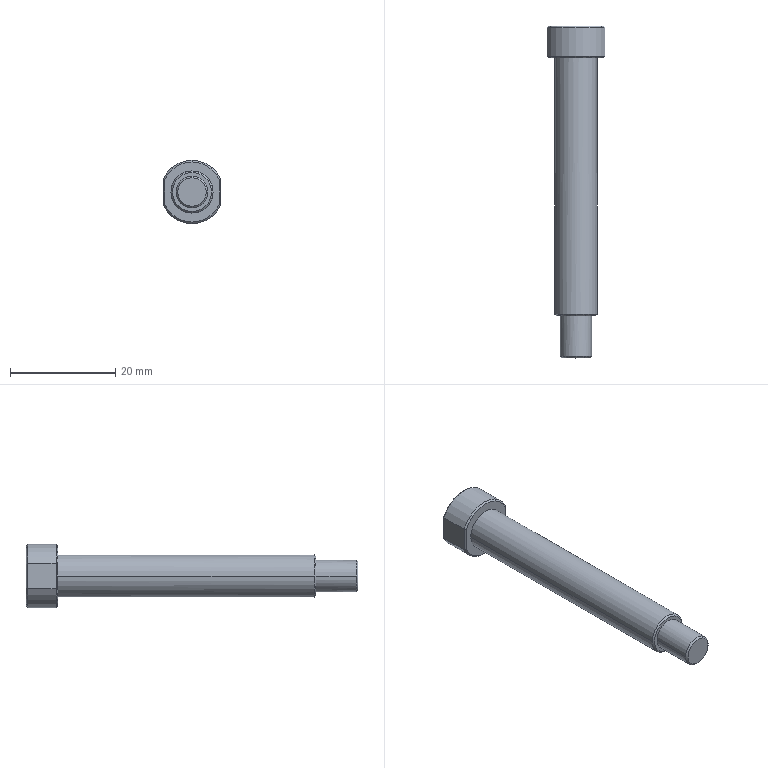Component | SolidWorks | LH-CGJ-01-058-2 | 1 solid | 26 faces | box 11 x 63 x 12 mm | volume 3343 mm3 | cone 10 | plane 10 | cylinder 6 | commonest cylinder face diameters 8 x2 6 x2 12 x2 | material #45
build123d program:
from build123d import *

# Parameters (mm, degrees)
CUT_EXTRUDE1_DEPTH = 59.558
CHAMFER1_SIZE      = 0.3


with BuildPart() as part:
    # Sketch1 → Revolve2 (revolve)
    with BuildSketch(Plane.XY, mode=Mode.PRIVATE) as revolve2_sk:
        Polygon((0, 0), (6, 0), (6, -63), (3, -63), (3, -55), (2, -55), (2, -6), (0, -6), align=None)
    revolve(revolve2_sk.sketch.rotate(Axis((6, -63, 0), (0, 1, 0)), 180), axis=Axis((6, -63, 0), (0, 1, 0)))

    # Sketch2 → Cut-Extrude1 (cut, through all)
    with BuildSketch(Plane.XZ.offset(6)):
        with BuildLine():
            Line((0.5, 2.398), (0.5, -2.398))
            ThreePointArc((0.5, -2.398), (0, 0), (0.5, 2.398))
        make_face()
        with BuildLine():
            Line((11.5, 2.398), (11.5, -2.398))
            ThreePointArc((11.5, -2.398), (12, 0), (11.5, 2.398))
        make_face()
    extrude(amount=-CUT_EXTRUDE1_DEPTH, mode=Mode.SUBTRACT)

    # Chamfer1
    chamfer1_edges = [part.edges().sort_by_distance(p)[0] for p in [
        (6, -6, -6),
        (6, 0, -6),
        (11.5, 0, 0),
        (11.5, -6, 0),
        (0.5, 0, 0),
        (0.5, -6, 0),
        (6, -6, 6),
        (2, -55, 0),
        (3, -63, 0),
        (6, 0, 6),
    ]]
    chamfer(chamfer1_edges, length=CHAMFER1_SIZE)


solid = part.part

# Placed as in the assembly
solid = solid.moved(Location((-42.003, 46.715, 115.05), (0, 0, 0)))
STEP:
#1=COLOUR_RGB('',0.7922,0.8196,0.9333);
#2=FILL_AREA_STYLE_COLOUR('',#1);
#3=FILL_AREA_STYLE('',(#2));
#4=SURFACE_STYLE_FILL_AREA(#3);
#5=SURFACE_SIDE_STYLE('',(#4));
#6=SURFACE_STYLE_USAGE(.BOTH.,#5);
#7=PRESENTATION_STYLE_ASSIGNMENT((#6));
#8=CARTESIAN_POINT('',(-1.417,-0.3262,4.384));
#9=VERTEX_POINT('',#8);
#10=CARTESIAN_POINT('',(-1.417,-0.3262,4.675));
#11=VERTEX_POINT('',#10);
#12=CARTESIAN_POINT('',(-1.417,-0.3262,4.53));
#13=DIRECTION('',(-0.,-1.,0.));
#14=DIRECTION('',(-1.,0.,0.));
#15=AXIS2_PLACEMENT_3D('',#12,#13,#14);
#16=CIRCLE('',#15,0.1457);
#17=EDGE_CURVE('',#9,#11,#16,.T.);
#18=ORIENTED_EDGE('',*,*,#17,.F.);
#19=CARTESIAN_POINT('',(-1.417,-0.3144,4.372));
#20=VERTEX_POINT('',#19);
#21=CARTESIAN_POINT('',(-1.417,-0.3262,4.384));
#22=DIRECTION('',(0.,0.7071,-0.7071));
#23=VECTOR('',#22,39.37);
#24=LINE('',#21,#23);
#25=EDGE_CURVE('',#9,#20,#24,.T.);
#26=ORIENTED_EDGE('',*,*,#25,.T.);
#27=CARTESIAN_POINT('',(-1.26,-0.3144,4.53));
#28=VERTEX_POINT('',#27);
#29=CARTESIAN_POINT('',(-1.417,-0.3144,4.53));
#30=DIRECTION('',(0.,1.,0.));
#31=DIRECTION('',(0.,0.,1.));
#32=AXIS2_PLACEMENT_3D('',#29,#30,#31);
#33=CIRCLE('',#32,0.1575);
#34=EDGE_CURVE('',#28,#20,#33,.T.);
#35=ORIENTED_EDGE('',*,*,#34,.F.);
#36=CARTESIAN_POINT('',(-1.417,-0.3144,4.687));
#37=VERTEX_POINT('',#36);
#38=CARTESIAN_POINT('',(-1.417,-0.3144,4.53));
#39=DIRECTION('',(0.,1.,0.));
#40=DIRECTION('',(0.,0.,1.));
#41=AXIS2_PLACEMENT_3D('',#38,#39,#40);
#42=CIRCLE('',#41,0.1575);
#43=EDGE_CURVE('',#37,#28,#42,.T.);
#44=ORIENTED_EDGE('',*,*,#43,.F.);
#45=CARTESIAN_POINT('',(-1.417,-0.3262,4.675));
#46=DIRECTION('',(0.,0.7071,0.7071));
#47=VECTOR('',#46,39.37);
#48=LINE('',#45,#47);
#49=EDGE_CURVE('',#11,#37,#48,.T.);
#50=ORIENTED_EDGE('',*,*,#49,.F.);
#51=EDGE_LOOP('',(#18,#26,#35,#44,#50));
#52=FACE_OUTER_BOUND('',#51,.T.);
#53=CARTESIAN_POINT('',(-1.417,-0.3262,4.53));
#54=DIRECTION('',(0.,1.,0.));
#55=DIRECTION('',(0.,0.,1.));
#56=AXIS2_PLACEMENT_3D('',#53,#54,#55);
#57=CONICAL_SURFACE('',#56,0.1457,0.7854);
#58=ADVANCED_FACE('',(#52),#57,.T.);
#59=CARTESIAN_POINT('',(-1.417,-0.6411,4.423));
#60=VERTEX_POINT('',#59);
#61=CARTESIAN_POINT('',(-1.417,-0.6411,4.636));
#62=VERTEX_POINT('',#61);
#63=CARTESIAN_POINT('',(-1.417,-0.6411,4.53));
#64=DIRECTION('',(-0.,-1.,0.));
#65=DIRECTION('',(-1.,0.,0.));
#66=AXIS2_PLACEMENT_3D('',#63,#64,#65);
#67=CIRCLE('',#66,0.1063);
#68=EDGE_CURVE('',#60,#62,#67,.T.);
#69=ORIENTED_EDGE('',*,*,#68,.F.);
#70=CARTESIAN_POINT('',(-1.417,-0.6293,4.411));
#71=VERTEX_POINT('',#70);
#72=CARTESIAN_POINT('',(-1.417,-0.6411,4.423));
#73=DIRECTION('',(0.,0.7071,-0.7071));
#74=VECTOR('',#73,39.37);
#75=LINE('',#72,#74);
#76=EDGE_CURVE('',#60,#71,#75,.T.);
#77=ORIENTED_EDGE('',*,*,#76,.T.);
#78=CARTESIAN_POINT('',(-1.299,-0.6293,4.53));
#79=VERTEX_POINT('',#78);
#80=CARTESIAN_POINT('',(-1.417,-0.6293,4.53));
#81=DIRECTION('',(0.,1.,0.));
#82=DIRECTION('',(0.,0.,1.));
#83=AXIS2_PLACEMENT_3D('',#80,#81,#82);
#84=CIRCLE('',#83,0.1181);
#85=EDGE_CURVE('',#79,#71,#84,.T.);
#86=ORIENTED_EDGE('',*,*,#85,.F.);
#87=CARTESIAN_POINT('',(-1.417,-0.6293,4.648));
#88=VERTEX_POINT('',#87);
#89=CARTESIAN_POINT('',(-1.417,-0.6293,4.53));
#90=DIRECTION('',(0.,1.,0.));
#91=DIRECTION('',(0.,0.,1.));
#92=AXIS2_PLACEMENT_3D('',#89,#90,#91);
#93=CIRCLE('',#92,0.1181);
#94=EDGE_CURVE('',#88,#79,#93,.T.);
#95=ORIENTED_EDGE('',*,*,#94,.F.);
#96=CARTESIAN_POINT('',(-1.417,-0.6411,4.636));
#97=DIRECTION('',(0.,0.7071,0.7071));
#98=VECTOR('',#97,39.37);
#99=LINE('',#96,#98);
#100=EDGE_CURVE('',#62,#88,#99,.T.);
#101=ORIENTED_EDGE('',*,*,#100,.F.);
#102=EDGE_LOOP('',(#69,#77,#86,#95,#101));
#103=FACE_OUTER_BOUND('',#102,.T.);
#104=CARTESIAN_POINT('',(-1.417,-0.6411,4.53));
#105=DIRECTION('',(0.,1.,0.));
#106=DIRECTION('',(0.,0.,1.));
#107=AXIS2_PLACEMENT_3D('',#104,#105,#106);
#108=CONICAL_SURFACE('',#107,0.1063,0.7854);
#109=ADVANCED_FACE('',(#103),#108,.T.);
#110=CARTESIAN_POINT('',(-1.417,1.603,4.754));
#111=VERTEX_POINT('',#110);
#112=CARTESIAN_POINT('',(-1.622,1.603,4.621));
#113=VERTEX_POINT('',#112);
#114=CARTESIAN_POINT('',(-1.417,1.603,4.53));
#115=DIRECTION('',(-0.,-1.,0.));
#116=DIRECTION('',(-1.,0.,0.));
#117=AXIS2_PLACEMENT_3D('',#114,#115,#116);
#118=CIRCLE('',#117,0.2244);
#119=EDGE_CURVE('',#111,#113,#118,.T.);
#120=ORIENTED_EDGE('',*,*,#119,.F.);
#121=CARTESIAN_POINT('',(-1.417,1.615,4.766));
#122=VERTEX_POINT('',#121);
#123=CARTESIAN_POINT('',(-1.417,1.603,4.754));
#124=DIRECTION('',(0.,0.7071,0.7071));
#125=VECTOR('',#124,39.37);
#126=LINE('',#123,#125);
#127=EDGE_CURVE('',#111,#122,#126,.T.);
#128=ORIENTED_EDGE('',*,*,#127,.T.);
#129=CARTESIAN_POINT('',(-1.634,1.615,4.624));
#130=VERTEX_POINT('',#129);
#131=CARTESIAN_POINT('',(-1.417,1.615,4.53));
#132=DIRECTION('',(0.,1.,0.));
#133=DIRECTION('',(0.,0.,1.));
#134=AXIS2_PLACEMENT_3D('',#131,#132,#133);
#135=CIRCLE('',#134,0.2362);
#136=EDGE_CURVE('',#130,#122,#135,.T.);
#137=ORIENTED_EDGE('',*,*,#136,.F.);
#138=CARTESIAN_POINT('',(-1.634,1.615,4.624));
#139=CARTESIAN_POINT('',(-1.63,1.611,4.623));
#140=CARTESIAN_POINT('',(-1.626,1.607,4.622));
#141=CARTESIAN_POINT('',(-1.622,1.603,4.621));
#142=B_SPLINE_CURVE_WITH_KNOTS('',3,(#138,#139,#140,#141),.UNSPECIFIED.,.F.,.F.,(4,4),(0.,0.000429),.UNSPECIFIED.);
#143=EDGE_CURVE('',#130,#113,#142,.T.);
#144=ORIENTED_EDGE('',*,*,#143,.T.);
#145=EDGE_LOOP('',(#120,#128,#137,#144));
#146=FACE_OUTER_BOUND('',#145,.T.);
#147=CARTESIAN_POINT('',(-1.417,1.603,4.53));
#148=DIRECTION('',(0.,1.,0.));
#149=DIRECTION('',(0.,0.,1.));
#150=AXIS2_PLACEMENT_3D('',#147,#148,#149);
#151=CONICAL_SURFACE('',#150,0.2244,0.7854);
#152=ADVANCED_FACE('',(#146),#151,.T.);
#153=CARTESIAN_POINT('',(-1.417,1.839,4.305));
#154=VERTEX_POINT('',#153);
#155=CARTESIAN_POINT('',(-1.622,1.839,4.438));
#156=VERTEX_POINT('',#155);
#157=CARTESIAN_POINT('',(-1.417,1.839,4.53));
#158=DIRECTION('',(0.,1.,0.));
#159=DIRECTION('',(1.,0.,0.));
#160=AXIS2_PLACEMENT_3D('',#157,#158,#159);
#161=CIRCLE('',#160,0.2244);
#162=EDGE_CURVE('',#154,#156,#161,.T.);
#163=ORIENTED_EDGE('',*,*,#162,.F.);
#164=CARTESIAN_POINT('',(-1.417,1.827,4.293));
#165=VERTEX_POINT('',#164);
#166=CARTESIAN_POINT('',(-1.417,1.827,4.293));
#167=DIRECTION('',(0.,-0.7071,-0.7071));
#168=VECTOR('',#167,39.37);
#169=LINE('',#166,#168);
#170=EDGE_CURVE('',#154,#165,#169,.T.);
#171=ORIENTED_EDGE('',*,*,#170,.T.);
#172=CARTESIAN_POINT('',(-1.634,1.827,4.435));
#173=VERTEX_POINT('',#172);
#174=CARTESIAN_POINT('',(-1.417,1.827,4.53));
#175=DIRECTION('',(0.,-1.,0.));
#176=DIRECTION('',(0.,0.,-1.));
#177=AXIS2_PLACEMENT_3D('',#174,#175,#176);
#178=CIRCLE('',#177,0.2362);
#179=EDGE_CURVE('',#173,#165,#178,.T.);
#180=ORIENTED_EDGE('',*,*,#179,.F.);
#181=CARTESIAN_POINT('',(-1.622,1.839,4.438));
#182=CARTESIAN_POINT('',(-1.626,1.835,4.437));
#183=CARTESIAN_POINT('',(-1.63,1.831,4.436));
#184=CARTESIAN_POINT('',(-1.634,1.827,4.435));
#185=B_SPLINE_CURVE_WITH_KNOTS('',3,(#181,#182,#183,#184),.UNSPECIFIED.,.F.,.F.,(4,4),(0.,0.000429),.UNSPECIFIED.);
#186=EDGE_CURVE('',#156,#173,#185,.T.);
#187=ORIENTED_EDGE('',*,*,#186,.F.);
#188=EDGE_LOOP('',(#163,#171,#180,#187));
#189=FACE_OUTER_BOUND('',#188,.T.);
#190=CARTESIAN_POINT('',(-1.417,1.827,4.53));
#191=DIRECTION('',(0.,-1.,0.));
#192=DIRECTION('',(0.,0.,-1.));
#193=AXIS2_PLACEMENT_3D('',#190,#191,#192);
#194=CONICAL_SURFACE('',#193,0.2362,0.7854);
#195=ADVANCED_FACE('',(#189),#194,.T.);
#196=CARTESIAN_POINT('',(-1.26,1.603,4.53));
#197=VERTEX_POINT('',#196);
#198=CARTESIAN_POINT('',(-1.575,1.603,4.53));
#199=VERTEX_POINT('',#198);
#200=CARTESIAN_POINT('',(-1.417,1.603,4.53));
#201=DIRECTION('',(-0.,-1.,0.));
#202=DIRECTION('',(1.,0.,0.));
#203=AXIS2_PLACEMENT_3D('',#200,#201,#202);
#204=CIRCLE('',#203,0.1575);
#205=EDGE_CURVE('',#197,#199,#204,.T.);
#206=ORIENTED_EDGE('',*,*,#205,.T.);
#207=CARTESIAN_POINT('',(-1.575,-0.3144,4.53));
#208=VERTEX_POINT('',#207);
#209=CARTESIAN_POINT('',(-1.575,-0.6411,4.53));
#210=DIRECTION('',(-0.,-1.,0.));
#211=VECTOR('',#210,39.37);
#212=LINE('',#209,#211);
#213=EDGE_CURVE('',#199,#208,#212,.T.);
#214=ORIENTED_EDGE('',*,*,#213,.T.);
#215=CARTESIAN_POINT('',(-1.417,-0.3144,4.53));
#216=DIRECTION('',(0.,1.,0.));
#217=DIRECTION('',(0.,0.,1.));
#218=AXIS2_PLACEMENT_3D('',#215,#216,#217);
#219=CIRCLE('',#218,0.1575);
#220=EDGE_CURVE('',#208,#37,#219,.T.);
#221=ORIENTED_EDGE('',*,*,#220,.T.);
#222=ORIENTED_EDGE('',*,*,#43,.T.);
#223=CARTESIAN_POINT('',(-1.26,-0.6411,4.53));
#224=DIRECTION('',(-0.,-1.,0.));
#225=VECTOR('',#224,39.37);
#226=LINE('',#223,#225);
#227=EDGE_CURVE('',#197,#28,#226,.T.);
#228=ORIENTED_EDGE('',*,*,#227,.F.);
#229=EDGE_LOOP('',(#206,#214,#221,#222,#228));
#230=FACE_OUTER_BOUND('',#229,.T.);
#231=CARTESIAN_POINT('',(-1.417,-0.6411,4.53));
#232=DIRECTION('',(-0.,-1.,0.));
#233=DIRECTION('',(1.,0.,0.));
#234=AXIS2_PLACEMENT_3D('',#231,#232,#233);
#235=CYLINDRICAL_SURFACE('',#234,0.1575);
#236=ADVANCED_FACE('',(#230),#235,.T.);
#237=CARTESIAN_POINT('',(-1.299,-0.3262,4.53));
#238=VERTEX_POINT('',#237);
#239=CARTESIAN_POINT('',(-1.536,-0.3262,4.53));
#240=VERTEX_POINT('',#239);
#241=CARTESIAN_POINT('',(-1.417,-0.3262,4.53));
#242=DIRECTION('',(-0.,-1.,0.));
#243=DIRECTION('',(1.,0.,0.));
#244=AXIS2_PLACEMENT_3D('',#241,#242,#243);
#245=CIRCLE('',#244,0.1181);
#246=EDGE_CURVE('',#238,#240,#245,.T.);
#247=ORIENTED_EDGE('',*,*,#246,.T.);
#248=CARTESIAN_POINT('',(-1.536,-0.6293,4.53));
#249=VERTEX_POINT('',#248);
#250=CARTESIAN_POINT('',(-1.536,-0.6411,4.53));
#251=DIRECTION('',(-0.,-1.,0.));
#252=VECTOR('',#251,39.37);
#253=LINE('',#250,#252);
#254=EDGE_CURVE('',#240,#249,#253,.T.);
#255=ORIENTED_EDGE('',*,*,#254,.T.);
#256=CARTESIAN_POINT('',(-1.417,-0.6293,4.53));
#257=DIRECTION('',(0.,1.,0.));
#258=DIRECTION('',(0.,0.,1.));
#259=AXIS2_PLACEMENT_3D('',#256,#257,#258);
#260=CIRCLE('',#259,0.1181);
#261=EDGE_CURVE('',#249,#88,#260,.T.);
#262=ORIENTED_EDGE('',*,*,#261,.T.);
#263=ORIENTED_EDGE('',*,*,#94,.T.);
#264=CARTESIAN_POINT('',(-1.299,-0.6411,4.53));
#265=DIRECTION('',(-0.,-1.,0.));
#266=VECTOR('',#265,39.37);
#267=LINE('',#264,#266);
#268=EDGE_CURVE('',#238,#79,#267,.T.);
#269=ORIENTED_EDGE('',*,*,#268,.F.);
#270=EDGE_LOOP('',(#247,#255,#262,#263,#269));
#271=FACE_OUTER_BOUND('',#270,.T.);
#272=CARTESIAN_POINT('',(-1.417,-0.6411,4.53));
#273=DIRECTION('',(-0.,-1.,0.));
#274=DIRECTION('',(1.,0.,0.));
#275=AXIS2_PLACEMENT_3D('',#272,#273,#274);
#276=CYLINDRICAL_SURFACE('',#275,0.1181);
#277=ADVANCED_FACE('',(#271),#276,.T.);
#278=CARTESIAN_POINT('',(-1.634,1.615,4.435));
#279=VERTEX_POINT('',#278);
#280=CARTESIAN_POINT('',(-1.634,1.839,4.435));
#281=DIRECTION('',(0.,-1.,0.));
#282=VECTOR('',#281,39.37);
#283=LINE('',#280,#282);
#284=EDGE_CURVE('',#173,#279,#283,.T.);
#285=ORIENTED_EDGE('',*,*,#284,.F.);
#286=ORIENTED_EDGE('',*,*,#179,.T.);
#287=CARTESIAN_POINT('',(-1.201,1.827,4.435));
#288=VERTEX_POINT('',#287);
#289=CARTESIAN_POINT('',(-1.417,1.827,4.53));
#290=DIRECTION('',(0.,-1.,0.));
#291=DIRECTION('',(0.,0.,-1.));
#292=AXIS2_PLACEMENT_3D('',#289,#290,#291);
#293=CIRCLE('',#292,0.2362);
#294=EDGE_CURVE('',#165,#288,#293,.T.);
#295=ORIENTED_EDGE('',*,*,#294,.T.);
#296=CARTESIAN_POINT('',(-1.201,1.615,4.435));
#297=VERTEX_POINT('',#296);
#298=CARTESIAN_POINT('',(-1.201,1.839,4.435));
#299=DIRECTION('',(0.,-1.,0.));
#300=VECTOR('',#299,39.37);
#301=LINE('',#298,#300);
#302=EDGE_CURVE('',#288,#297,#301,.T.);
#303=ORIENTED_EDGE('',*,*,#302,.T.);
#304=CARTESIAN_POINT('',(-1.417,1.615,4.53));
#305=DIRECTION('',(0.,1.,0.));
#306=DIRECTION('',(0.,0.,1.));
#307=AXIS2_PLACEMENT_3D('',#304,#305,#306);
#308=CIRCLE('',#307,0.2362);
#309=EDGE_CURVE('',#297,#279,#308,.T.);
#310=ORIENTED_EDGE('',*,*,#309,.T.);
#311=EDGE_LOOP('',(#285,#286,#295,#303,#310));
#312=FACE_OUTER_BOUND('',#311,.T.);
#313=CARTESIAN_POINT('',(-1.417,-0.6411,4.53));
#314=DIRECTION('',(-0.,-1.,0.));
#315=DIRECTION('',(1.,0.,0.));
#316=AXIS2_PLACEMENT_3D('',#313,#314,#315);
#317=CYLINDRICAL_SURFACE('',#316,0.2362);
#318=ADVANCED_FACE('',(#312),#317,.T.);
#319=CARTESIAN_POINT('',(-1.201,1.827,4.624));
#320=VERTEX_POINT('',#319);
#321=CARTESIAN_POINT('',(-1.201,1.615,4.624));
#322=VERTEX_POINT('',#321);
#323=CARTESIAN_POINT('',(-1.201,1.839,4.624));
#324=DIRECTION('',(0.,-1.,0.));
#325=VECTOR('',#324,39.37);
#326=LINE('',#323,#325);
#327=EDGE_CURVE('',#320,#322,#326,.T.);
#328=ORIENTED_EDGE('',*,*,#327,.F.);
#329=CARTESIAN_POINT('',(-1.634,1.827,4.624));
#330=VERTEX_POINT('',#329);
#331=CARTESIAN_POINT('',(-1.417,1.827,4.53));
#332=DIRECTION('',(0.,-1.,0.));
#333=DIRECTION('',(0.,0.,-1.));
#334=AXIS2_PLACEMENT_3D('',#331,#332,#333);
#335=CIRCLE('',#334,0.2362);
#336=EDGE_CURVE('',#320,#330,#335,.T.);
#337=ORIENTED_EDGE('',*,*,#336,.T.);
#338=CARTESIAN_POINT('',(-1.634,1.839,4.624));
#339=DIRECTION('',(0.,-1.,0.));
#340=VECTOR('',#339,39.37);
#341=LINE('',#338,#340);
#342=EDGE_CURVE('',#330,#130,#341,.T.);
#343=ORIENTED_EDGE('',*,*,#342,.T.);
#344=ORIENTED_EDGE('',*,*,#136,.T.);
#345=CARTESIAN_POINT('',(-1.417,1.615,4.53));
#346=DIRECTION('',(0.,1.,0.));
#347=DIRECTION('',(0.,0.,1.));
#348=AXIS2_PLACEMENT_3D('',#345,#346,#347);
#349=CIRCLE('',#348,0.2362);
#350=EDGE_CURVE('',#122,#322,#349,.T.);
#351=ORIENTED_EDGE('',*,*,#350,.T.);
#352=EDGE_LOOP('',(#328,#337,#343,#344,#351));
#353=FACE_OUTER_BOUND('',#352,.T.);
#354=CARTESIAN_POINT('',(-1.417,-0.6411,4.53));
#355=DIRECTION('',(-0.,-1.,0.));
#356=DIRECTION('',(1.,0.,0.));
#357=AXIS2_PLACEMENT_3D('',#354,#355,#356);
#358=CYLINDRICAL_SURFACE('',#357,0.2362);
#359=ADVANCED_FACE('',(#353),#358,.T.);
#360=CARTESIAN_POINT('',(-1.622,1.839,4.621));
#361=VERTEX_POINT('',#360);
#362=CARTESIAN_POINT('',(-1.622,1.839,4.53));
#363=DIRECTION('',(0.,0.,1.));
#364=VECTOR('',#363,39.37);
#365=LINE('',#362,#364);
#366=EDGE_CURVE('',#156,#361,#365,.T.);
#367=ORIENTED_EDGE('',*,*,#366,.T.);
#368=CARTESIAN_POINT('',(-1.213,1.839,4.621));
#369=VERTEX_POINT('',#368);
#370=CARTESIAN_POINT('',(-1.417,1.839,4.53));
#371=DIRECTION('',(0.,1.,0.));
#372=DIRECTION('',(1.,0.,0.));
#373=AXIS2_PLACEMENT_3D('',#370,#371,#372);
#374=CIRCLE('',#373,0.2244);
#375=EDGE_CURVE('',#361,#369,#374,.T.);
#376=ORIENTED_EDGE('',*,*,#375,.T.);
#377=CARTESIAN_POINT('',(-1.213,1.839,4.438));
#378=VERTEX_POINT('',#377);
#379=CARTESIAN_POINT('',(-1.213,1.839,4.53));
#380=DIRECTION('',(0.,0.,-1.));
#381=VECTOR('',#380,39.37);
#382=LINE('',#379,#381);
#383=EDGE_CURVE('',#369,#378,#382,.T.);
#384=ORIENTED_EDGE('',*,*,#383,.T.);
#385=CARTESIAN_POINT('',(-1.417,1.839,4.53));
#386=DIRECTION('',(0.,1.,0.));
#387=DIRECTION('',(1.,0.,0.));
#388=AXIS2_PLACEMENT_3D('',#385,#386,#387);
#389=CIRCLE('',#388,0.2244);
#390=EDGE_CURVE('',#378,#154,#389,.T.);
#391=ORIENTED_EDGE('',*,*,#390,.T.);
#392=ORIENTED_EDGE('',*,*,#162,.T.);
#393=EDGE_LOOP('',(#367,#376,#384,#391,#392));
#394=FACE_OUTER_BOUND('',#393,.T.);
#395=CARTESIAN_POINT('',(-1.654,1.839,4.53));
#396=DIRECTION('',(-0.,-1.,0.));
#397=DIRECTION('',(1.,-0.,0.));
#398=AXIS2_PLACEMENT_3D('',#395,#396,#397);
#399=PLANE('',#398);
#400=ADVANCED_FACE('',(#394),#399,.F.);
#401=CARTESIAN_POINT('',(-1.417,-0.6411,4.53));
#402=DIRECTION('',(-0.,-1.,0.));
#403=DIRECTION('',(-1.,0.,0.));
#404=AXIS2_PLACEMENT_3D('',#401,#402,#403);
#405=CIRCLE('',#404,0.1063);
#406=EDGE_CURVE('',#62,#60,#405,.T.);
#407=ORIENTED_EDGE('',*,*,#406,.T.);
#408=ORIENTED_EDGE('',*,*,#68,.T.);
#409=EDGE_LOOP('',(#407,#408));
#410=FACE_OUTER_BOUND('',#409,.T.);
#411=CARTESIAN_POINT('',(-1.417,-0.6411,4.53));
#412=DIRECTION('',(0.,1.,0.));
#413=DIRECTION('',(-1.,0.,0.));
#414=AXIS2_PLACEMENT_3D('',#411,#412,#413);
#415=PLANE('',#414);
#416=ADVANCED_FACE('',(#410),#415,.F.);
#417=ORIENTED_EDGE('',*,*,#254,.F.);
#418=CARTESIAN_POINT('',(-1.417,-0.3262,4.53));
#419=DIRECTION('',(-0.,-1.,0.));
#420=DIRECTION('',(1.,0.,0.));
#421=AXIS2_PLACEMENT_3D('',#418,#419,#420);
#422=CIRCLE('',#421,0.1181);
#423=EDGE_CURVE('',#240,#238,#422,.T.);
#424=ORIENTED_EDGE('',*,*,#423,.T.);
#425=ORIENTED_EDGE('',*,*,#268,.T.);
#426=ORIENTED_EDGE('',*,*,#85,.T.);
#427=CARTESIAN_POINT('',(-1.417,-0.6293,4.53));
#428=DIRECTION('',(0.,1.,0.));
#429=DIRECTION('',(0.,0.,1.));
#430=AXIS2_PLACEMENT_3D('',#427,#428,#429);
#431=CIRCLE('',#430,0.1181);
#432=EDGE_CURVE('',#71,#249,#431,.T.);
#433=ORIENTED_EDGE('',*,*,#432,.T.);
#434=EDGE_LOOP('',(#417,#424,#425,#426,#433));
#435=FACE_OUTER_BOUND('',#434,.T.);
#436=CARTESIAN_POINT('',(-1.417,-0.6411,4.53));
#437=DIRECTION('',(-0.,-1.,0.));
#438=DIRECTION('',(1.,0.,0.));
#439=AXIS2_PLACEMENT_3D('',#436,#437,#438);
#440=CYLINDRICAL_SURFACE('',#439,0.1181);
#441=ADVANCED_FACE('',(#435),#440,.T.);
#442=CARTESIAN_POINT('',(-1.417,-0.3262,4.53));
#443=DIRECTION('',(-0.,-1.,0.));
#444=DIRECTION('',(-1.,0.,0.));
#445=AXIS2_PLACEMENT_3D('',#442,#443,#444);
#446=CIRCLE('',#445,0.1457);
#447=EDGE_CURVE('',#11,#9,#446,.T.);
#448=ORIENTED_EDGE('',*,*,#447,.T.);
#449=ORIENTED_EDGE('',*,*,#17,.T.);
#450=EDGE_LOOP('',(#448,#449));
#451=FACE_OUTER_BOUND('',#450,.T.);
#452=ORIENTED_EDGE('',*,*,#246,.F.);
#453=ORIENTED_EDGE('',*,*,#423,.F.);
#454=EDGE_LOOP('',(#452,#453));
#455=FACE_BOUND('',#454,.T.);
#456=CARTESIAN_POINT('',(-1.575,-0.3262,4.53));
#457=DIRECTION('',(0.,1.,0.));
#458=DIRECTION('',(-1.,0.,0.));
#459=AXIS2_PLACEMENT_3D('',#456,#457,#458);
#460=PLANE('',#459);
#461=ADVANCED_FACE('',(#451,#455),#460,.F.);
#462=ORIENTED_EDGE('',*,*,#213,.F.);
#463=CARTESIAN_POINT('',(-1.417,1.603,4.53));
#464=DIRECTION('',(-0.,-1.,0.));
#465=DIRECTION('',(1.,0.,0.));
#466=AXIS2_PLACEMENT_3D('',#463,#464,#465);
#467=CIRCLE('',#466,0.1575);
#468=EDGE_CURVE('',#199,#197,#467,.T.);
#469=ORIENTED_EDGE('',*,*,#468,.T.);
#470=ORIENTED_EDGE('',*,*,#227,.T.);
#471=ORIENTED_EDGE('',*,*,#34,.T.);
#472=CARTESIAN_POINT('',(-1.417,-0.3144,4.53));
#473=DIRECTION('',(0.,1.,0.));
#474=DIRECTION('',(0.,0.,1.));
#475=AXIS2_PLACEMENT_3D('',#472,#473,#474);
#476=CIRCLE('',#475,0.1575);
#477=EDGE_CURVE('',#20,#208,#476,.T.);
#478=ORIENTED_EDGE('',*,*,#477,.T.);
#479=EDGE_LOOP('',(#462,#469,#470,#471,#478));
#480=FACE_OUTER_BOUND('',#479,.T.);
#481=CARTESIAN_POINT('',(-1.417,-0.6411,4.53));
#482=DIRECTION('',(-0.,-1.,0.));
#483=DIRECTION('',(1.,0.,0.));
#484=AXIS2_PLACEMENT_3D('',#481,#482,#483);
#485=CYLINDRICAL_SURFACE('',#484,0.1575);
#486=ADVANCED_FACE('',(#480),#485,.T.);
#487=CARTESIAN_POINT('',(-1.622,1.603,4.438));
#488=VERTEX_POINT('',#487);
#489=CARTESIAN_POINT('',(-1.213,1.603,4.438));
#490=VERTEX_POINT('',#489);
#491=CARTESIAN_POINT('',(-1.417,1.603,4.53));
#492=DIRECTION('',(-0.,-1.,0.));
#493=DIRECTION('',(-1.,0.,0.));
#494=AXIS2_PLACEMENT_3D('',#491,#492,#493);
#495=CIRCLE('',#494,0.2244);
#496=EDGE_CURVE('',#488,#490,#495,.T.);
#497=ORIENTED_EDGE('',*,*,#496,.T.);
#498=CARTESIAN_POINT('',(-1.213,1.603,4.621));
#499=VERTEX_POINT('',#498);
#500=CARTESIAN_POINT('',(-1.213,1.603,4.53));
#501=DIRECTION('',(0.,0.,1.));
#502=VECTOR('',#501,39.37);
#503=LINE('',#500,#502);
#504=EDGE_CURVE('',#490,#499,#503,.T.);
#505=ORIENTED_EDGE('',*,*,#504,.T.);
#506=CARTESIAN_POINT('',(-1.417,1.603,4.53));
#507=DIRECTION('',(-0.,-1.,0.));
#508=DIRECTION('',(-1.,0.,-0.));
#509=AXIS2_PLACEMENT_3D('',#506,#507,#508);
#510=CIRCLE('',#509,0.2244);
#511=EDGE_CURVE('',#499,#111,#510,.T.);
#512=ORIENTED_EDGE('',*,*,#511,.T.);
#513=ORIENTED_EDGE('',*,*,#119,.T.);
#514=CARTESIAN_POINT('',(-1.622,1.603,4.53));
#515=DIRECTION('',(0.,0.,-1.));
#516=VECTOR('',#515,39.37);
#517=LINE('',#514,#516);
#518=EDGE_CURVE('',#113,#488,#517,.T.);
#519=ORIENTED_EDGE('',*,*,#518,.T.);
#520=EDGE_LOOP('',(#497,#505,#512,#513,#519));
#521=FACE_OUTER_BOUND('',#520,.T.);
#522=ORIENTED_EDGE('',*,*,#205,.F.);
#523=ORIENTED_EDGE('',*,*,#468,.F.);
#524=EDGE_LOOP('',(#522,#523));
#525=FACE_BOUND('',#524,.T.);
#526=CARTESIAN_POINT('',(-1.575,1.603,4.53));
#527=DIRECTION('',(0.,1.,0.));
#528=DIRECTION('',(-1.,0.,0.));
#529=AXIS2_PLACEMENT_3D('',#526,#527,#528);
#530=PLANE('',#529);
#531=ADVANCED_FACE('',(#521,#525),#530,.F.);
#532=ORIENTED_EDGE('',*,*,#342,.F.);
#533=CARTESIAN_POINT('',(-1.634,1.827,4.624));
#534=DIRECTION('',(0.,0.,-1.));
#535=VECTOR('',#534,39.37);
#536=LINE('',#533,#535);
#537=EDGE_CURVE('',#330,#173,#536,.T.);
#538=ORIENTED_EDGE('',*,*,#537,.T.);
#539=ORIENTED_EDGE('',*,*,#284,.T.);
#540=CARTESIAN_POINT('',(-1.634,1.615,4.624));
#541=DIRECTION('',(0.,0.,1.));
#542=VECTOR('',#541,39.37);
#543=LINE('',#540,#542);
#544=EDGE_CURVE('',#279,#130,#543,.T.);
#545=ORIENTED_EDGE('',*,*,#544,.T.);
#546=EDGE_LOOP('',(#532,#538,#539,#545));
#547=FACE_OUTER_BOUND('',#546,.T.);
#548=CARTESIAN_POINT('',(-1.634,1.839,4.624));
#549=DIRECTION('',(1.,0.,0.));
#550=DIRECTION('',(-0.,1.,0.));
#551=AXIS2_PLACEMENT_3D('',#548,#549,#550);
#552=PLANE('',#551);
#553=ADVANCED_FACE('',(#547),#552,.F.);
#554=ORIENTED_EDGE('',*,*,#302,.F.);
#555=CARTESIAN_POINT('',(-1.201,1.827,4.624));
#556=DIRECTION('',(0.,0.,1.));
#557=VECTOR('',#556,39.37);
#558=LINE('',#555,#557);
#559=EDGE_CURVE('',#288,#320,#558,.T.);
#560=ORIENTED_EDGE('',*,*,#559,.T.);
#561=ORIENTED_EDGE('',*,*,#327,.T.);
#562=CARTESIAN_POINT('',(-1.201,1.615,4.624));
#563=DIRECTION('',(0.,0.,-1.));
#564=VECTOR('',#563,39.37);
#565=LINE('',#562,#564);
#566=EDGE_CURVE('',#322,#297,#565,.T.);
#567=ORIENTED_EDGE('',*,*,#566,.T.);
#568=EDGE_LOOP('',(#554,#560,#561,#567));
#569=FACE_OUTER_BOUND('',#568,.T.);
#570=CARTESIAN_POINT('',(-1.201,1.839,4.624));
#571=DIRECTION('',(-1.,-0.,0.));
#572=DIRECTION('',(0.,-1.,0.));
#573=AXIS2_PLACEMENT_3D('',#570,#571,#572);
#574=PLANE('',#573);
#575=ADVANCED_FACE('',(#569),#574,.F.);
#576=ORIENTED_EDGE('',*,*,#170,.F.);
#577=ORIENTED_EDGE('',*,*,#390,.F.);
#578=CARTESIAN_POINT('',(-1.201,1.827,4.435));
#579=CARTESIAN_POINT('',(-1.205,1.831,4.436));
#580=CARTESIAN_POINT('',(-1.209,1.835,4.437));
#581=CARTESIAN_POINT('',(-1.213,1.839,4.438));
#582=B_SPLINE_CURVE_WITH_KNOTS('',3,(#578,#579,#580,#581),.UNSPECIFIED.,.F.,.F.,(4,4),(0.,0.000429),.UNSPECIFIED.);
#583=EDGE_CURVE('',#288,#378,#582,.T.);
#584=ORIENTED_EDGE('',*,*,#583,.F.);
#585=ORIENTED_EDGE('',*,*,#294,.F.);
#586=EDGE_LOOP('',(#576,#577,#584,#585));
#587=FACE_OUTER_BOUND('',#586,.T.);
#588=CARTESIAN_POINT('',(-1.417,1.827,4.53));
#589=DIRECTION('',(0.,-1.,0.));
#590=DIRECTION('',(0.,0.,-1.));
#591=AXIS2_PLACEMENT_3D('',#588,#589,#590);
#592=CONICAL_SURFACE('',#591,0.2362,0.7854);
#593=ADVANCED_FACE('',(#587),#592,.T.);
#594=ORIENTED_EDGE('',*,*,#583,.T.);
#595=ORIENTED_EDGE('',*,*,#383,.F.);
#596=CARTESIAN_POINT('',(-1.201,1.827,4.624));
#597=CARTESIAN_POINT('',(-1.205,1.831,4.623));
#598=CARTESIAN_POINT('',(-1.209,1.835,4.622));
#599=CARTESIAN_POINT('',(-1.213,1.839,4.621));
#600=B_SPLINE_CURVE_WITH_KNOTS('',3,(#596,#597,#598,#599),.UNSPECIFIED.,.F.,.F.,(4,4),(0.,0.000429),.UNSPECIFIED.);
#601=EDGE_CURVE('',#320,#369,#600,.T.);
#602=ORIENTED_EDGE('',*,*,#601,.F.);
#603=ORIENTED_EDGE('',*,*,#559,.F.);
#604=EDGE_LOOP('',(#594,#595,#602,#603));
#605=FACE_OUTER_BOUND('',#604,.T.);
#606=CARTESIAN_POINT('',(-1.213,1.839,4.53));
#607=DIRECTION('',(-0.7071,-0.7071,0.));
#608=DIRECTION('',(0.,0.,-1.));
#609=AXIS2_PLACEMENT_3D('',#606,#607,#608);
#610=PLANE('',#609);
#611=ADVANCED_FACE('',(#605),#610,.F.);
#612=ORIENTED_EDGE('',*,*,#186,.T.);
#613=ORIENTED_EDGE('',*,*,#537,.F.);
#614=CARTESIAN_POINT('',(-1.622,1.839,4.621));
#615=CARTESIAN_POINT('',(-1.626,1.835,4.622));
#616=CARTESIAN_POINT('',(-1.63,1.831,4.623));
#617=CARTESIAN_POINT('',(-1.634,1.827,4.624));
#618=B_SPLINE_CURVE_WITH_KNOTS('',3,(#614,#615,#616,#617),.UNSPECIFIED.,.F.,.F.,(4,4),(0.,0.000429),.UNSPECIFIED.);
#619=EDGE_CURVE('',#361,#330,#618,.T.);
#620=ORIENTED_EDGE('',*,*,#619,.F.);
#621=ORIENTED_EDGE('',*,*,#366,.F.);
#622=EDGE_LOOP('',(#612,#613,#620,#621));
#623=FACE_OUTER_BOUND('',#622,.T.);
#624=CARTESIAN_POINT('',(-1.622,1.839,4.53));
#625=DIRECTION('',(0.7071,-0.7071,0.));
#626=DIRECTION('',(0.,0.,1.));
#627=AXIS2_PLACEMENT_3D('',#624,#625,#626);
#628=PLANE('',#627);
#629=ADVANCED_FACE('',(#623),#628,.F.);
#630=ORIENTED_EDGE('',*,*,#601,.T.);
#631=ORIENTED_EDGE('',*,*,#375,.F.);
#632=ORIENTED_EDGE('',*,*,#619,.T.);
#633=ORIENTED_EDGE('',*,*,#336,.F.);
#634=EDGE_LOOP('',(#630,#631,#632,#633));
#635=FACE_OUTER_BOUND('',#634,.T.);
#636=CARTESIAN_POINT('',(-1.417,1.827,4.53));
#637=DIRECTION('',(0.,-1.,0.));
#638=DIRECTION('',(0.,0.,-1.));
#639=AXIS2_PLACEMENT_3D('',#636,#637,#638);
#640=CONICAL_SURFACE('',#639,0.2362,0.7854);
#641=ADVANCED_FACE('',(#635),#640,.T.);
#642=CARTESIAN_POINT('',(-1.622,1.603,4.438));
#643=CARTESIAN_POINT('',(-1.626,1.607,4.437));
#644=CARTESIAN_POINT('',(-1.63,1.611,4.436));
#645=CARTESIAN_POINT('',(-1.634,1.615,4.435));
#646=B_SPLINE_CURVE_WITH_KNOTS('',3,(#642,#643,#644,#645),.UNSPECIFIED.,.F.,.F.,(4,4),(0.,0.000429),.UNSPECIFIED.);
#647=EDGE_CURVE('',#488,#279,#646,.T.);
#648=ORIENTED_EDGE('',*,*,#647,.F.);
#649=ORIENTED_EDGE('',*,*,#518,.F.);
#650=ORIENTED_EDGE('',*,*,#143,.F.);
#651=ORIENTED_EDGE('',*,*,#544,.F.);
#652=EDGE_LOOP('',(#648,#649,#650,#651));
#653=FACE_OUTER_BOUND('',#652,.T.);
#654=CARTESIAN_POINT('',(-1.634,1.615,4.624));
#655=DIRECTION('',(0.7071,0.7071,0.));
#656=DIRECTION('',(0.,0.,1.));
#657=AXIS2_PLACEMENT_3D('',#654,#655,#656);
#658=PLANE('',#657);
#659=ADVANCED_FACE('',(#653),#658,.F.);
#660=ORIENTED_EDGE('',*,*,#127,.F.);
#661=ORIENTED_EDGE('',*,*,#511,.F.);
#662=CARTESIAN_POINT('',(-1.201,1.615,4.624));
#663=CARTESIAN_POINT('',(-1.205,1.611,4.623));
#664=CARTESIAN_POINT('',(-1.209,1.607,4.622));
#665=CARTESIAN_POINT('',(-1.213,1.603,4.621));
#666=B_SPLINE_CURVE_WITH_KNOTS('',3,(#662,#663,#664,#665),.UNSPECIFIED.,.F.,.F.,(4,4),(0.,0.000429),.UNSPECIFIED.);
#667=EDGE_CURVE('',#322,#499,#666,.T.);
#668=ORIENTED_EDGE('',*,*,#667,.F.);
#669=ORIENTED_EDGE('',*,*,#350,.F.);
#670=EDGE_LOOP('',(#660,#661,#668,#669));
#671=FACE_OUTER_BOUND('',#670,.T.);
#672=CARTESIAN_POINT('',(-1.417,1.603,4.53));
#673=DIRECTION('',(0.,1.,0.));
#674=DIRECTION('',(0.,0.,1.));
#675=AXIS2_PLACEMENT_3D('',#672,#673,#674);
#676=CONICAL_SURFACE('',#675,0.2244,0.7854);
#677=ADVANCED_FACE('',(#671),#676,.T.);
#678=ORIENTED_EDGE('',*,*,#647,.T.);
#679=ORIENTED_EDGE('',*,*,#309,.F.);
#680=CARTESIAN_POINT('',(-1.213,1.603,4.438));
#681=CARTESIAN_POINT('',(-1.209,1.607,4.437));
#682=CARTESIAN_POINT('',(-1.205,1.611,4.436));
#683=CARTESIAN_POINT('',(-1.201,1.615,4.435));
#684=B_SPLINE_CURVE_WITH_KNOTS('',3,(#680,#681,#682,#683),.UNSPECIFIED.,.F.,.F.,(4,4),(0.,0.000429),.UNSPECIFIED.);
#685=EDGE_CURVE('',#490,#297,#684,.T.);
#686=ORIENTED_EDGE('',*,*,#685,.F.);
#687=ORIENTED_EDGE('',*,*,#496,.F.);
#688=EDGE_LOOP('',(#678,#679,#686,#687));
#689=FACE_OUTER_BOUND('',#688,.T.);
#690=CARTESIAN_POINT('',(-1.417,1.603,4.53));
#691=DIRECTION('',(0.,1.,0.));
#692=DIRECTION('',(0.,0.,1.));
#693=AXIS2_PLACEMENT_3D('',#690,#691,#692);
#694=CONICAL_SURFACE('',#693,0.2244,0.7854);
#695=ADVANCED_FACE('',(#689),#694,.T.);
#696=ORIENTED_EDGE('',*,*,#667,.T.);
#697=ORIENTED_EDGE('',*,*,#504,.F.);
#698=ORIENTED_EDGE('',*,*,#685,.T.);
#699=ORIENTED_EDGE('',*,*,#566,.F.);
#700=EDGE_LOOP('',(#696,#697,#698,#699));
#701=FACE_OUTER_BOUND('',#700,.T.);
#702=CARTESIAN_POINT('',(-1.201,1.615,4.624));
#703=DIRECTION('',(-0.7071,0.7071,0.));
#704=DIRECTION('',(0.,0.,-1.));
#705=AXIS2_PLACEMENT_3D('',#702,#703,#704);
#706=PLANE('',#705);
#707=ADVANCED_FACE('',(#701),#706,.F.);
#708=ORIENTED_EDGE('',*,*,#76,.F.);
#709=ORIENTED_EDGE('',*,*,#406,.F.);
#710=ORIENTED_EDGE('',*,*,#100,.T.);
#711=ORIENTED_EDGE('',*,*,#261,.F.);
#712=ORIENTED_EDGE('',*,*,#432,.F.);
#713=EDGE_LOOP('',(#708,#709,#710,#711,#712));
#714=FACE_OUTER_BOUND('',#713,.T.);
#715=CARTESIAN_POINT('',(-1.417,-0.6411,4.53));
#716=DIRECTION('',(0.,1.,0.));
#717=DIRECTION('',(0.,0.,1.));
#718=AXIS2_PLACEMENT_3D('',#715,#716,#717);
#719=CONICAL_SURFACE('',#718,0.1063,0.7854);
#720=ADVANCED_FACE('',(#714),#719,.T.);
#721=ORIENTED_EDGE('',*,*,#25,.F.);
#722=ORIENTED_EDGE('',*,*,#447,.F.);
#723=ORIENTED_EDGE('',*,*,#49,.T.);
#724=ORIENTED_EDGE('',*,*,#220,.F.);
#725=ORIENTED_EDGE('',*,*,#477,.F.);
#726=EDGE_LOOP('',(#721,#722,#723,#724,#725));
#727=FACE_OUTER_BOUND('',#726,.T.);
#728=CARTESIAN_POINT('',(-1.417,-0.3262,4.53));
#729=DIRECTION('',(0.,1.,0.));
#730=DIRECTION('',(0.,0.,1.));
#731=AXIS2_PLACEMENT_3D('',#728,#729,#730);
#732=CONICAL_SURFACE('',#731,0.1457,0.7854);
#733=ADVANCED_FACE('',(#727),#732,.T.);
#734=CLOSED_SHELL('',(#58,#109,#152,#195,#236,#277,#318,#359,#400,#416,#441,#461,#486,#531,#553,#575,#593,#611,#629,#641,#659,#677,#695,#707,#720,#733));
#735=MANIFOLD_SOLID_BREP('',#734);
#736=STYLED_ITEM('',(#7),#735);
#737=PRESENTATION_LAYER_ASSIGNMENT('','',(#736));
#738=CARTESIAN_POINT('',(0.,0.,0.));
#739=DIRECTION('',(0.,0.,1.));
#740=DIRECTION('',(1.,0.,0.));
#741=AXIS2_PLACEMENT_3D('',#738,#739,#740);
#742=(LENGTH_UNIT()NAMED_UNIT(*)SI_UNIT($,.METRE.));
#743=LENGTH_MEASURE_WITH_UNIT(LENGTH_MEASURE(0.0254),#742);
#744=DIMENSIONAL_EXPONENTS(1.,0.,0.,0.,0.,0.,0.);
#745=(CONVERSION_BASED_UNIT('',#743)LENGTH_UNIT()NAMED_UNIT(#744));
#746=UNCERTAINTY_MEASURE_WITH_UNIT(LENGTH_MEASURE(0.00001),#745,'','');
#747=(NAMED_UNIT(*)PLANE_ANGLE_UNIT()SI_UNIT($,.RADIAN.));
#748=(NAMED_UNIT(*)SI_UNIT($,.STERADIAN.)SOLID_ANGLE_UNIT());
#749=(GEOMETRIC_REPRESENTATION_CONTEXT(3)GLOBAL_UNCERTAINTY_ASSIGNED_CONTEXT((#746))GLOBAL_UNIT_ASSIGNED_CONTEXT((#745,#747,#748))REPRESENTATION_CONTEXT('',''));
#750=ADVANCED_BREP_SHAPE_REPRESENTATION('',(#735,#741),#749);
#751=(LENGTH_UNIT()NAMED_UNIT(*)SI_UNIT($,.METRE.));
#752=LENGTH_MEASURE_WITH_UNIT(LENGTH_MEASURE(0.0254),#751);
#753=DIMENSIONAL_EXPONENTS(1.,0.,0.,0.,0.,0.,0.);
#754=(CONVERSION_BASED_UNIT('',#752)LENGTH_UNIT()NAMED_UNIT(#753));
#755=UNCERTAINTY_MEASURE_WITH_UNIT(LENGTH_MEASURE(0.00001),#754,'','');
#756=(NAMED_UNIT(*)PLANE_ANGLE_UNIT()SI_UNIT($,.RADIAN.));
#757=(NAMED_UNIT(*)SI_UNIT($,.STERADIAN.)SOLID_ANGLE_UNIT());
#758=(GEOMETRIC_REPRESENTATION_CONTEXT(3)GLOBAL_UNCERTAINTY_ASSIGNED_CONTEXT((#755))GLOBAL_UNIT_ASSIGNED_CONTEXT((#754,#756,#757))REPRESENTATION_CONTEXT('',''));
#759=MECHANICAL_DESIGN_GEOMETRIC_PRESENTATION_REPRESENTATION('',(#736),#758);